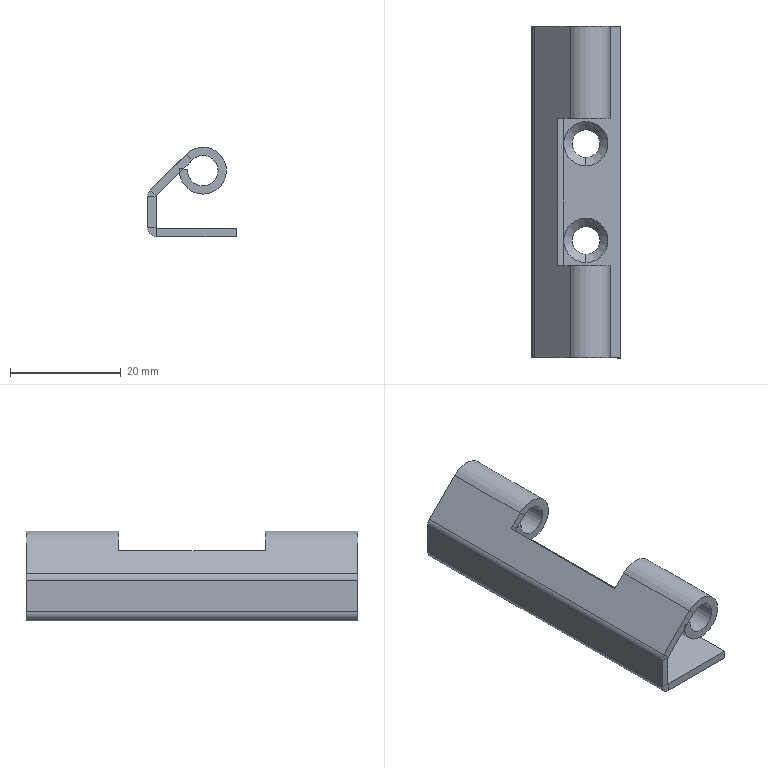Component | SolidWorks | AEBox-BoxHinge-3 | 1 solid | 38 faces | box 16 x 60 x 16.21 mm | volume 3571 mm3 | plane 26 | cylinder 8 | cone 4 | commonest cylinder face diameters 3.2 x2 0.2 x2 8.5 x2 5.5 x2
STEP:
#1=COLOUR_RGB('',0.7922,0.8196,0.9333);
#2=FILL_AREA_STYLE_COLOUR('',#1);
#3=FILL_AREA_STYLE('',(#2));
#4=SURFACE_STYLE_FILL_AREA(#3);
#5=SURFACE_SIDE_STYLE('',(#4));
#6=SURFACE_STYLE_USAGE(.BOTH.,#5);
#7=PRESENTATION_STYLE_ASSIGNMENT((#6));
#8=CARTESIAN_POINT('',(9.75,-14.031,37.663));
#9=VERTEX_POINT('',#8);
#10=CARTESIAN_POINT('',(9.75,-14.228,37.663));
#11=VERTEX_POINT('',#10);
#12=CARTESIAN_POINT('',(9.75,-14.129,37.663));
#13=DIRECTION('',(-0.,0.,-1.));
#14=DIRECTION('',(0.,-1.,0.));
#15=AXIS2_PLACEMENT_3D('',#12,#13,#14);
#16=CIRCLE('',#15,0.09843);
#17=EDGE_CURVE('',#9,#11,#16,.T.);
#18=ORIENTED_EDGE('',*,*,#17,.T.);
#19=CARTESIAN_POINT('',(9.75,-14.287,37.722));
#20=VERTEX_POINT('',#19);
#21=CARTESIAN_POINT('',(9.75,-14.287,37.722));
#22=DIRECTION('',(-0.,-0.7071,0.7071));
#23=VECTOR('',#22,39.37);
#24=LINE('',#21,#23);
#25=EDGE_CURVE('',#11,#20,#24,.T.);
#26=ORIENTED_EDGE('',*,*,#25,.T.);
#27=CARTESIAN_POINT('',(9.75,-13.972,37.722));
#28=VERTEX_POINT('',#27);
#29=CARTESIAN_POINT('',(9.75,-14.129,37.722));
#30=DIRECTION('',(-0.,0.,-1.));
#31=DIRECTION('',(-0.,-1.,0.));
#32=AXIS2_PLACEMENT_3D('',#29,#30,#31);
#33=CIRCLE('',#32,0.1575);
#34=EDGE_CURVE('',#28,#20,#33,.T.);
#35=ORIENTED_EDGE('',*,*,#34,.F.);
#36=CARTESIAN_POINT('',(9.75,-13.972,37.722));
#37=DIRECTION('',(0.,0.7071,0.7071));
#38=VECTOR('',#37,39.37);
#39=LINE('',#36,#38);
#40=EDGE_CURVE('',#9,#28,#39,.T.);
#41=ORIENTED_EDGE('',*,*,#40,.F.);
#42=EDGE_LOOP('',(#18,#26,#35,#41));
#43=FACE_OUTER_BOUND('',#42,.T.);
#44=CARTESIAN_POINT('',(9.75,-14.129,37.722));
#45=DIRECTION('',(0.,-0.,1.));
#46=DIRECTION('',(0.,1.,0.));
#47=AXIS2_PLACEMENT_3D('',#44,#45,#46);
#48=CONICAL_SURFACE('',#47,0.1575,0.7854);
#49=ADVANCED_FACE('',(#43),#48,.F.);
#50=CARTESIAN_POINT('',(9.75,-13.342,37.663));
#51=VERTEX_POINT('',#50);
#52=CARTESIAN_POINT('',(9.75,-13.539,37.663));
#53=VERTEX_POINT('',#52);
#54=CARTESIAN_POINT('',(9.75,-13.44,37.663));
#55=DIRECTION('',(-0.,0.,-1.));
#56=DIRECTION('',(0.,-1.,0.));
#57=AXIS2_PLACEMENT_3D('',#54,#55,#56);
#58=CIRCLE('',#57,0.09843);
#59=EDGE_CURVE('',#51,#53,#58,.T.);
#60=ORIENTED_EDGE('',*,*,#59,.T.);
#61=CARTESIAN_POINT('',(9.75,-13.598,37.722));
#62=VERTEX_POINT('',#61);
#63=CARTESIAN_POINT('',(9.75,-13.598,37.722));
#64=DIRECTION('',(-0.,-0.7071,0.7071));
#65=VECTOR('',#64,39.37);
#66=LINE('',#63,#65);
#67=EDGE_CURVE('',#53,#62,#66,.T.);
#68=ORIENTED_EDGE('',*,*,#67,.T.);
#69=CARTESIAN_POINT('',(9.75,-13.283,37.722));
#70=VERTEX_POINT('',#69);
#71=CARTESIAN_POINT('',(9.75,-13.44,37.722));
#72=DIRECTION('',(-0.,0.,-1.));
#73=DIRECTION('',(-0.,-1.,0.));
#74=AXIS2_PLACEMENT_3D('',#71,#72,#73);
#75=CIRCLE('',#74,0.1575);
#76=EDGE_CURVE('',#70,#62,#75,.T.);
#77=ORIENTED_EDGE('',*,*,#76,.F.);
#78=CARTESIAN_POINT('',(9.75,-13.283,37.722));
#79=DIRECTION('',(0.,0.7071,0.7071));
#80=VECTOR('',#79,39.37);
#81=LINE('',#78,#80);
#82=EDGE_CURVE('',#51,#70,#81,.T.);
#83=ORIENTED_EDGE('',*,*,#82,.F.);
#84=EDGE_LOOP('',(#60,#68,#77,#83));
#85=FACE_OUTER_BOUND('',#84,.T.);
#86=CARTESIAN_POINT('',(9.75,-13.44,37.722));
#87=DIRECTION('',(0.,-0.,1.));
#88=DIRECTION('',(0.,1.,0.));
#89=AXIS2_PLACEMENT_3D('',#86,#87,#88);
#90=CONICAL_SURFACE('',#89,0.1575,0.7854);
#91=ADVANCED_FACE('',(#85),#90,.F.);
#92=CARTESIAN_POINT('',(9.68,-14.966,38.21));
#93=VERTEX_POINT('',#92);
#94=CARTESIAN_POINT('',(9.424,-14.966,37.955));
#95=VERTEX_POINT('',#94);
#96=CARTESIAN_POINT('',(9.423,-14.966,37.953));
#97=DIRECTION('',(-0.7071,0.,-0.7071));
#98=VECTOR('',#97,39.37);
#99=LINE('',#96,#98);
#100=EDGE_CURVE('',#93,#95,#99,.T.);
#101=ORIENTED_EDGE('',*,*,#100,.F.);
#102=CARTESIAN_POINT('',(9.638,-14.966,38.252));
#103=VERTEX_POINT('',#102);
#104=CARTESIAN_POINT('',(9.68,-14.966,38.21));
#105=DIRECTION('',(-0.7071,0.,0.7071));
#106=VECTOR('',#105,39.37);
#107=LINE('',#104,#106);
#108=EDGE_CURVE('',#93,#103,#107,.T.);
#109=ORIENTED_EDGE('',*,*,#108,.T.);
#110=CARTESIAN_POINT('',(9.382,-14.966,37.996));
#111=VERTEX_POINT('',#110);
#112=CARTESIAN_POINT('',(9.381,-14.966,37.995));
#113=DIRECTION('',(-0.7071,0.,-0.7071));
#114=VECTOR('',#113,39.37);
#115=LINE('',#112,#114);
#116=EDGE_CURVE('',#103,#111,#115,.T.);
#117=ORIENTED_EDGE('',*,*,#116,.T.);
#118=CARTESIAN_POINT('',(9.424,-14.966,37.955));
#119=DIRECTION('',(-0.7071,0.,0.7071));
#120=VECTOR('',#119,39.37);
#121=LINE('',#118,#120);
#122=EDGE_CURVE('',#95,#111,#121,.T.);
#123=ORIENTED_EDGE('',*,*,#122,.F.);
#124=EDGE_LOOP('',(#101,#109,#117,#123));
#125=FACE_OUTER_BOUND('',#124,.T.);
#126=CARTESIAN_POINT('',(9.381,-14.966,37.995));
#127=DIRECTION('',(-0.,-1.,-0.));
#128=DIRECTION('',(0.,-0.,1.));
#129=AXIS2_PLACEMENT_3D('',#126,#127,#128);
#130=PLANE('',#129);
#131=ADVANCED_FACE('',(#125),#130,.T.);
#132=CARTESIAN_POINT('',(9.423,-14.966,37.952));
#133=VERTEX_POINT('',#132);
#134=CARTESIAN_POINT('',(9.364,-14.966,37.952));
#135=VERTEX_POINT('',#134);
#136=CARTESIAN_POINT('',(9.423,-14.966,37.952));
#137=DIRECTION('',(-1.,0.,0.));
#138=VECTOR('',#137,39.37);
#139=LINE('',#136,#138);
#140=EDGE_CURVE('',#133,#135,#139,.T.);
#141=ORIENTED_EDGE('',*,*,#140,.T.);
#142=CARTESIAN_POINT('',(9.364,-14.966,37.726));
#143=VERTEX_POINT('',#142);
#144=CARTESIAN_POINT('',(9.364,-14.966,37.722));
#145=DIRECTION('',(-0.,-0.,1.));
#146=VECTOR('',#145,39.37);
#147=LINE('',#144,#146);
#148=EDGE_CURVE('',#143,#135,#147,.T.);
#149=ORIENTED_EDGE('',*,*,#148,.F.);
#150=CARTESIAN_POINT('',(9.423,-14.966,37.726));
#151=VERTEX_POINT('',#150);
#152=CARTESIAN_POINT('',(9.423,-14.966,37.726));
#153=DIRECTION('',(-1.,0.,-0.));
#154=VECTOR('',#153,39.37);
#155=LINE('',#152,#154);
#156=EDGE_CURVE('',#151,#143,#155,.T.);
#157=ORIENTED_EDGE('',*,*,#156,.F.);
#158=CARTESIAN_POINT('',(9.423,-14.966,37.978));
#159=DIRECTION('',(-0.,-0.,1.));
#160=VECTOR('',#159,39.37);
#161=LINE('',#158,#160);
#162=EDGE_CURVE('',#151,#133,#161,.T.);
#163=ORIENTED_EDGE('',*,*,#162,.T.);
#164=EDGE_LOOP('',(#141,#149,#157,#163));
#165=FACE_OUTER_BOUND('',#164,.T.);
#166=CARTESIAN_POINT('',(9.364,-14.966,37.978));
#167=DIRECTION('',(0.,1.,0.));
#168=DIRECTION('',(-0.,0.,-1.));
#169=AXIS2_PLACEMENT_3D('',#166,#167,#168);
#170=PLANE('',#169);
#171=ADVANCED_FACE('',(#165),#170,.F.);
#172=CARTESIAN_POINT('',(9.423,-12.604,37.952));
#173=VERTEX_POINT('',#172);
#174=CARTESIAN_POINT('',(9.364,-12.604,37.952));
#175=VERTEX_POINT('',#174);
#176=CARTESIAN_POINT('',(9.423,-12.604,37.952));
#177=DIRECTION('',(-1.,0.,0.));
#178=VECTOR('',#177,39.37);
#179=LINE('',#176,#178);
#180=EDGE_CURVE('',#173,#175,#179,.T.);
#181=ORIENTED_EDGE('',*,*,#180,.F.);
#182=CARTESIAN_POINT('',(9.423,-12.604,37.726));
#183=VERTEX_POINT('',#182);
#184=CARTESIAN_POINT('',(9.423,-12.604,37.722));
#185=DIRECTION('',(0.,0.,-1.));
#186=VECTOR('',#185,39.37);
#187=LINE('',#184,#186);
#188=EDGE_CURVE('',#173,#183,#187,.T.);
#189=ORIENTED_EDGE('',*,*,#188,.T.);
#190=CARTESIAN_POINT('',(9.364,-12.604,37.726));
#191=VERTEX_POINT('',#190);
#192=CARTESIAN_POINT('',(9.364,-12.604,37.726));
#193=DIRECTION('',(-1.,0.,-0.));
#194=VECTOR('',#193,39.37);
#195=LINE('',#192,#194);
#196=EDGE_CURVE('',#183,#191,#195,.T.);
#197=ORIENTED_EDGE('',*,*,#196,.T.);
#198=CARTESIAN_POINT('',(9.364,-12.604,37.722));
#199=DIRECTION('',(0.,0.,-1.));
#200=VECTOR('',#199,39.37);
#201=LINE('',#198,#200);
#202=EDGE_CURVE('',#175,#191,#201,.T.);
#203=ORIENTED_EDGE('',*,*,#202,.F.);
#204=EDGE_LOOP('',(#181,#189,#197,#203));
#205=FACE_OUTER_BOUND('',#204,.T.);
#206=CARTESIAN_POINT('',(9.364,-12.604,37.722));
#207=DIRECTION('',(-0.,-1.,-0.));
#208=DIRECTION('',(0.,-0.,1.));
#209=AXIS2_PLACEMENT_3D('',#206,#207,#208);
#210=PLANE('',#209);
#211=ADVANCED_FACE('',(#205),#210,.F.);
#212=CARTESIAN_POINT('',(9.364,-14.966,37.952));
#213=DIRECTION('',(0.,1.,0.));
#214=VECTOR('',#213,39.37);
#215=LINE('',#212,#214);
#216=EDGE_CURVE('',#135,#175,#215,.T.);
#217=ORIENTED_EDGE('',*,*,#216,.T.);
#218=ORIENTED_EDGE('',*,*,#202,.T.);
#219=CARTESIAN_POINT('',(9.364,-12.604,37.726));
#220=DIRECTION('',(0.,1.,0.));
#221=VECTOR('',#220,39.37);
#222=LINE('',#219,#221);
#223=EDGE_CURVE('',#143,#191,#222,.T.);
#224=ORIENTED_EDGE('',*,*,#223,.F.);
#225=ORIENTED_EDGE('',*,*,#148,.T.);
#226=EDGE_LOOP('',(#217,#218,#224,#225));
#227=FACE_OUTER_BOUND('',#226,.T.);
#228=CARTESIAN_POINT('',(9.364,-14.966,37.722));
#229=DIRECTION('',(1.,-0.,0.));
#230=DIRECTION('',(-0.,-0.,1.));
#231=AXIS2_PLACEMENT_3D('',#228,#229,#230);
#232=PLANE('',#231);
#233=ADVANCED_FACE('',(#227),#232,.F.);
#234=ORIENTED_EDGE('',*,*,#188,.F.);
#235=CARTESIAN_POINT('',(9.423,-14.966,37.952));
#236=DIRECTION('',(0.,1.,0.));
#237=VECTOR('',#236,39.37);
#238=LINE('',#235,#237);
#239=EDGE_CURVE('',#133,#173,#238,.T.);
#240=ORIENTED_EDGE('',*,*,#239,.F.);
#241=ORIENTED_EDGE('',*,*,#162,.F.);
#242=CARTESIAN_POINT('',(9.423,-12.604,37.726));
#243=DIRECTION('',(-0.,-1.,-0.));
#244=VECTOR('',#243,39.37);
#245=LINE('',#242,#244);
#246=EDGE_CURVE('',#183,#151,#245,.T.);
#247=ORIENTED_EDGE('',*,*,#246,.F.);
#248=EDGE_LOOP('',(#234,#240,#241,#247));
#249=FACE_OUTER_BOUND('',#248,.T.);
#250=CARTESIAN_POINT('',(9.423,-14.966,37.722));
#251=DIRECTION('',(1.,-0.,0.));
#252=DIRECTION('',(-0.,-0.,1.));
#253=AXIS2_PLACEMENT_3D('',#250,#251,#252);
#254=PLANE('',#253);
#255=ADVANCED_FACE('',(#249),#254,.T.);
#256=CARTESIAN_POINT('',(9.994,-14.966,37.722));
#257=VERTEX_POINT('',#256);
#258=CARTESIAN_POINT('',(9.427,-14.966,37.722));
#259=VERTEX_POINT('',#258);
#260=CARTESIAN_POINT('',(9.364,-14.966,37.722));
#261=DIRECTION('',(-1.,0.,0.));
#262=VECTOR('',#261,39.37);
#263=LINE('',#260,#262);
#264=EDGE_CURVE('',#257,#259,#263,.T.);
#265=ORIENTED_EDGE('',*,*,#264,.T.);
#266=CARTESIAN_POINT('',(9.427,-14.966,37.663));
#267=VERTEX_POINT('',#266);
#268=CARTESIAN_POINT('',(9.427,-14.966,37.722));
#269=DIRECTION('',(-0.,0.,-1.));
#270=VECTOR('',#269,39.37);
#271=LINE('',#268,#270);
#272=EDGE_CURVE('',#259,#267,#271,.T.);
#273=ORIENTED_EDGE('',*,*,#272,.T.);
#274=CARTESIAN_POINT('',(9.994,-14.966,37.663));
#275=VERTEX_POINT('',#274);
#276=CARTESIAN_POINT('',(9.364,-14.966,37.663));
#277=DIRECTION('',(-1.,0.,0.));
#278=VECTOR('',#277,39.37);
#279=LINE('',#276,#278);
#280=EDGE_CURVE('',#275,#267,#279,.T.);
#281=ORIENTED_EDGE('',*,*,#280,.F.);
#282=CARTESIAN_POINT('',(9.994,-14.966,37.722));
#283=DIRECTION('',(-0.,0.,-1.));
#284=VECTOR('',#283,39.37);
#285=LINE('',#282,#284);
#286=EDGE_CURVE('',#257,#275,#285,.T.);
#287=ORIENTED_EDGE('',*,*,#286,.F.);
#288=EDGE_LOOP('',(#265,#273,#281,#287));
#289=FACE_OUTER_BOUND('',#288,.T.);
#290=CARTESIAN_POINT('',(9.364,-14.966,37.722));
#291=DIRECTION('',(-0.,-1.,-0.));
#292=DIRECTION('',(-1.,0.,0.));
#293=AXIS2_PLACEMENT_3D('',#290,#291,#292);
#294=PLANE('',#293);
#295=ADVANCED_FACE('',(#289),#294,.T.);
#296=ORIENTED_EDGE('',*,*,#76,.T.);
#297=CARTESIAN_POINT('',(9.75,-13.44,37.722));
#298=DIRECTION('',(-0.,0.,-1.));
#299=DIRECTION('',(-0.,-1.,0.));
#300=AXIS2_PLACEMENT_3D('',#297,#298,#299);
#301=CIRCLE('',#300,0.1575);
#302=EDGE_CURVE('',#62,#70,#301,.T.);
#303=ORIENTED_EDGE('',*,*,#302,.T.);
#304=EDGE_LOOP('',(#296,#303));
#305=FACE_BOUND('',#304,.T.);
#306=ORIENTED_EDGE('',*,*,#34,.T.);
#307=CARTESIAN_POINT('',(9.75,-14.129,37.722));
#308=DIRECTION('',(-0.,0.,-1.));
#309=DIRECTION('',(-0.,-1.,0.));
#310=AXIS2_PLACEMENT_3D('',#307,#308,#309);
#311=CIRCLE('',#310,0.1575);
#312=EDGE_CURVE('',#20,#28,#311,.T.);
#313=ORIENTED_EDGE('',*,*,#312,.T.);
#314=EDGE_LOOP('',(#306,#313));
#315=FACE_BOUND('',#314,.T.);
#316=CARTESIAN_POINT('',(9.427,-12.604,37.722));
#317=VERTEX_POINT('',#316);
#318=CARTESIAN_POINT('',(9.427,-14.966,37.722));
#319=DIRECTION('',(0.,1.,0.));
#320=VECTOR('',#319,39.37);
#321=LINE('',#318,#320);
#322=EDGE_CURVE('',#259,#317,#321,.T.);
#323=ORIENTED_EDGE('',*,*,#322,.F.);
#324=ORIENTED_EDGE('',*,*,#264,.F.);
#325=CARTESIAN_POINT('',(9.994,-12.604,37.722));
#326=VERTEX_POINT('',#325);
#327=CARTESIAN_POINT('',(9.994,-12.604,37.722));
#328=DIRECTION('',(-0.,-1.,-0.));
#329=VECTOR('',#328,39.37);
#330=LINE('',#327,#329);
#331=EDGE_CURVE('',#326,#257,#330,.T.);
#332=ORIENTED_EDGE('',*,*,#331,.F.);
#333=CARTESIAN_POINT('',(9.364,-12.604,37.722));
#334=DIRECTION('',(1.,-0.,-0.));
#335=VECTOR('',#334,39.37);
#336=LINE('',#333,#335);
#337=EDGE_CURVE('',#317,#326,#336,.T.);
#338=ORIENTED_EDGE('',*,*,#337,.F.);
#339=EDGE_LOOP('',(#323,#324,#332,#338));
#340=FACE_OUTER_BOUND('',#339,.T.);
#341=CARTESIAN_POINT('',(9.994,-14.966,37.722));
#342=DIRECTION('',(-0.,0.,-1.));
#343=DIRECTION('',(-0.,-1.,-0.));
#344=AXIS2_PLACEMENT_3D('',#341,#342,#343);
#345=PLANE('',#344);
#346=ADVANCED_FACE('',(#305,#315,#340),#345,.F.);
#347=ORIENTED_EDGE('',*,*,#59,.F.);
#348=CARTESIAN_POINT('',(9.75,-13.44,37.663));
#349=DIRECTION('',(-0.,0.,-1.));
#350=DIRECTION('',(0.,-1.,0.));
#351=AXIS2_PLACEMENT_3D('',#348,#349,#350);
#352=CIRCLE('',#351,0.09843);
#353=EDGE_CURVE('',#53,#51,#352,.T.);
#354=ORIENTED_EDGE('',*,*,#353,.F.);
#355=EDGE_LOOP('',(#347,#354));
#356=FACE_BOUND('',#355,.T.);
#357=ORIENTED_EDGE('',*,*,#17,.F.);
#358=CARTESIAN_POINT('',(9.75,-14.129,37.663));
#359=DIRECTION('',(-0.,0.,-1.));
#360=DIRECTION('',(0.,-1.,0.));
#361=AXIS2_PLACEMENT_3D('',#358,#359,#360);
#362=CIRCLE('',#361,0.09843);
#363=EDGE_CURVE('',#11,#9,#362,.T.);
#364=ORIENTED_EDGE('',*,*,#363,.F.);
#365=EDGE_LOOP('',(#357,#364));
#366=FACE_BOUND('',#365,.T.);
#367=ORIENTED_EDGE('',*,*,#280,.T.);
#368=CARTESIAN_POINT('',(9.427,-12.604,37.663));
#369=VERTEX_POINT('',#368);
#370=CARTESIAN_POINT('',(9.427,-14.966,37.663));
#371=DIRECTION('',(0.,1.,0.));
#372=VECTOR('',#371,39.37);
#373=LINE('',#370,#372);
#374=EDGE_CURVE('',#267,#369,#373,.T.);
#375=ORIENTED_EDGE('',*,*,#374,.T.);
#376=CARTESIAN_POINT('',(9.994,-12.604,37.663));
#377=VERTEX_POINT('',#376);
#378=CARTESIAN_POINT('',(9.364,-12.604,37.663));
#379=DIRECTION('',(1.,-0.,-0.));
#380=VECTOR('',#379,39.37);
#381=LINE('',#378,#380);
#382=EDGE_CURVE('',#369,#377,#381,.T.);
#383=ORIENTED_EDGE('',*,*,#382,.T.);
#384=CARTESIAN_POINT('',(9.994,-12.604,37.663));
#385=DIRECTION('',(-0.,-1.,-0.));
#386=VECTOR('',#385,39.37);
#387=LINE('',#384,#386);
#388=EDGE_CURVE('',#377,#275,#387,.T.);
#389=ORIENTED_EDGE('',*,*,#388,.T.);
#390=EDGE_LOOP('',(#367,#375,#383,#389));
#391=FACE_OUTER_BOUND('',#390,.T.);
#392=CARTESIAN_POINT('',(9.994,-14.966,37.663));
#393=DIRECTION('',(-0.,0.,-1.));
#394=DIRECTION('',(-0.,-1.,-0.));
#395=AXIS2_PLACEMENT_3D('',#392,#393,#394);
#396=PLANE('',#395);
#397=ADVANCED_FACE('',(#356,#366,#391),#396,.T.);
#398=ORIENTED_EDGE('',*,*,#388,.F.);
#399=CARTESIAN_POINT('',(9.994,-12.604,37.722));
#400=DIRECTION('',(-0.,0.,-1.));
#401=VECTOR('',#400,39.37);
#402=LINE('',#399,#401);
#403=EDGE_CURVE('',#326,#377,#402,.T.);
#404=ORIENTED_EDGE('',*,*,#403,.F.);
#405=ORIENTED_EDGE('',*,*,#331,.T.);
#406=ORIENTED_EDGE('',*,*,#286,.T.);
#407=EDGE_LOOP('',(#398,#404,#405,#406));
#408=FACE_OUTER_BOUND('',#407,.T.);
#409=CARTESIAN_POINT('',(9.994,-12.604,37.722));
#410=DIRECTION('',(1.,-0.,-0.));
#411=DIRECTION('',(0.,-0.,1.));
#412=AXIS2_PLACEMENT_3D('',#409,#410,#411);
#413=PLANE('',#412);
#414=ADVANCED_FACE('',(#408),#413,.T.);
#415=CARTESIAN_POINT('',(9.427,-12.604,37.722));
#416=DIRECTION('',(-0.,0.,-1.));
#417=VECTOR('',#416,39.37);
#418=LINE('',#415,#417);
#419=EDGE_CURVE('',#317,#369,#418,.T.);
#420=ORIENTED_EDGE('',*,*,#419,.F.);
#421=ORIENTED_EDGE('',*,*,#337,.T.);
#422=ORIENTED_EDGE('',*,*,#403,.T.);
#423=ORIENTED_EDGE('',*,*,#382,.F.);
#424=EDGE_LOOP('',(#420,#421,#422,#423));
#425=FACE_OUTER_BOUND('',#424,.T.);
#426=CARTESIAN_POINT('',(9.364,-12.604,37.722));
#427=DIRECTION('',(0.,1.,0.));
#428=DIRECTION('',(1.,-0.,-0.));
#429=AXIS2_PLACEMENT_3D('',#426,#427,#428);
#430=PLANE('',#429);
#431=ADVANCED_FACE('',(#425),#430,.T.);
#432=ORIENTED_EDGE('',*,*,#196,.F.);
#433=CARTESIAN_POINT('',(9.427,-12.604,37.726));
#434=DIRECTION('',(0.,1.,0.));
#435=DIRECTION('',(0.,0.,1.));
#436=AXIS2_PLACEMENT_3D('',#433,#434,#435);
#437=CIRCLE('',#436,0.003937);
#438=EDGE_CURVE('',#317,#183,#437,.T.);
#439=ORIENTED_EDGE('',*,*,#438,.F.);
#440=ORIENTED_EDGE('',*,*,#419,.T.);
#441=CARTESIAN_POINT('',(9.427,-12.604,37.726));
#442=DIRECTION('',(0.,1.,0.));
#443=DIRECTION('',(0.,0.,1.));
#444=AXIS2_PLACEMENT_3D('',#441,#442,#443);
#445=CIRCLE('',#444,0.06299);
#446=EDGE_CURVE('',#369,#191,#445,.T.);
#447=ORIENTED_EDGE('',*,*,#446,.T.);
#448=EDGE_LOOP('',(#432,#439,#440,#447));
#449=FACE_OUTER_BOUND('',#448,.T.);
#450=CARTESIAN_POINT('',(9.427,-12.604,37.726));
#451=DIRECTION('',(0.,1.,0.));
#452=DIRECTION('',(-0.,0.,-1.));
#453=AXIS2_PLACEMENT_3D('',#450,#451,#452);
#454=PLANE('',#453);
#455=ADVANCED_FACE('',(#449),#454,.T.);
#456=CARTESIAN_POINT('',(9.427,-14.966,37.726));
#457=DIRECTION('',(-0.,-1.,-0.));
#458=DIRECTION('',(0.,0.,1.));
#459=AXIS2_PLACEMENT_3D('',#456,#457,#458);
#460=CIRCLE('',#459,0.003937);
#461=EDGE_CURVE('',#151,#259,#460,.T.);
#462=ORIENTED_EDGE('',*,*,#461,.F.);
#463=ORIENTED_EDGE('',*,*,#156,.T.);
#464=CARTESIAN_POINT('',(9.427,-14.966,37.726));
#465=DIRECTION('',(-0.,-1.,-0.));
#466=DIRECTION('',(0.,0.,1.));
#467=AXIS2_PLACEMENT_3D('',#464,#465,#466);
#468=CIRCLE('',#467,0.06299);
#469=EDGE_CURVE('',#143,#267,#468,.T.);
#470=ORIENTED_EDGE('',*,*,#469,.T.);
#471=ORIENTED_EDGE('',*,*,#272,.F.);
#472=EDGE_LOOP('',(#462,#463,#470,#471));
#473=FACE_OUTER_BOUND('',#472,.T.);
#474=CARTESIAN_POINT('',(9.427,-14.966,37.726));
#475=DIRECTION('',(0.,1.,0.));
#476=DIRECTION('',(-0.,0.,-1.));
#477=AXIS2_PLACEMENT_3D('',#474,#475,#476);
#478=PLANE('',#477);
#479=ADVANCED_FACE('',(#473),#478,.F.);
#480=ORIENTED_EDGE('',*,*,#374,.F.);
#481=ORIENTED_EDGE('',*,*,#469,.F.);
#482=ORIENTED_EDGE('',*,*,#223,.T.);
#483=ORIENTED_EDGE('',*,*,#446,.F.);
#484=EDGE_LOOP('',(#480,#481,#482,#483));
#485=FACE_OUTER_BOUND('',#484,.T.);
#486=CARTESIAN_POINT('',(9.427,-14.966,37.726));
#487=DIRECTION('',(-0.,-1.,-0.));
#488=DIRECTION('',(-1.,0.,0.));
#489=AXIS2_PLACEMENT_3D('',#486,#487,#488);
#490=CYLINDRICAL_SURFACE('',#489,0.06299);
#491=ADVANCED_FACE('',(#485),#490,.T.);
#492=ORIENTED_EDGE('',*,*,#322,.T.);
#493=ORIENTED_EDGE('',*,*,#438,.T.);
#494=ORIENTED_EDGE('',*,*,#246,.T.);
#495=ORIENTED_EDGE('',*,*,#461,.T.);
#496=EDGE_LOOP('',(#492,#493,#494,#495));
#497=FACE_OUTER_BOUND('',#496,.T.);
#498=CARTESIAN_POINT('',(9.427,-14.966,37.726));
#499=DIRECTION('',(-0.,-1.,-0.));
#500=DIRECTION('',(-1.,0.,0.));
#501=AXIS2_PLACEMENT_3D('',#498,#499,#500);
#502=CYLINDRICAL_SURFACE('',#501,0.003937);
#503=ADVANCED_FACE('',(#497),#502,.F.);
#504=CARTESIAN_POINT('',(9.424,-12.604,37.955));
#505=VERTEX_POINT('',#504);
#506=CARTESIAN_POINT('',(9.382,-12.604,37.996));
#507=VERTEX_POINT('',#506);
#508=CARTESIAN_POINT('',(9.382,-12.604,37.996));
#509=DIRECTION('',(-0.7071,0.,0.7071));
#510=VECTOR('',#509,39.37);
#511=LINE('',#508,#510);
#512=EDGE_CURVE('',#505,#507,#511,.T.);
#513=ORIENTED_EDGE('',*,*,#512,.F.);
#514=CARTESIAN_POINT('',(9.427,-12.604,37.952));
#515=DIRECTION('',(0.,1.,0.));
#516=DIRECTION('',(0.,0.,1.));
#517=AXIS2_PLACEMENT_3D('',#514,#515,#516);
#518=CIRCLE('',#517,0.003937);
#519=EDGE_CURVE('',#173,#505,#518,.T.);
#520=ORIENTED_EDGE('',*,*,#519,.F.);
#521=ORIENTED_EDGE('',*,*,#180,.T.);
#522=CARTESIAN_POINT('',(9.427,-12.604,37.952));
#523=DIRECTION('',(0.,1.,0.));
#524=DIRECTION('',(0.,0.,1.));
#525=AXIS2_PLACEMENT_3D('',#522,#523,#524);
#526=CIRCLE('',#525,0.06299);
#527=EDGE_CURVE('',#175,#507,#526,.T.);
#528=ORIENTED_EDGE('',*,*,#527,.T.);
#529=EDGE_LOOP('',(#513,#520,#521,#528));
#530=FACE_OUTER_BOUND('',#529,.T.);
#531=CARTESIAN_POINT('',(9.427,-12.604,37.952));
#532=DIRECTION('',(0.,1.,0.));
#533=DIRECTION('',(-0.,0.,-1.));
#534=AXIS2_PLACEMENT_3D('',#531,#532,#533);
#535=PLANE('',#534);
#536=ADVANCED_FACE('',(#530),#535,.T.);
#537=CARTESIAN_POINT('',(9.427,-14.966,37.952));
#538=DIRECTION('',(-0.,-1.,-0.));
#539=DIRECTION('',(0.,0.,1.));
#540=AXIS2_PLACEMENT_3D('',#537,#538,#539);
#541=CIRCLE('',#540,0.003937);
#542=EDGE_CURVE('',#95,#133,#541,.T.);
#543=ORIENTED_EDGE('',*,*,#542,.F.);
#544=ORIENTED_EDGE('',*,*,#122,.T.);
#545=CARTESIAN_POINT('',(9.427,-14.966,37.952));
#546=DIRECTION('',(-0.,-1.,-0.));
#547=DIRECTION('',(0.,0.,1.));
#548=AXIS2_PLACEMENT_3D('',#545,#546,#547);
#549=CIRCLE('',#548,0.06299);
#550=EDGE_CURVE('',#111,#135,#549,.T.);
#551=ORIENTED_EDGE('',*,*,#550,.T.);
#552=ORIENTED_EDGE('',*,*,#140,.F.);
#553=EDGE_LOOP('',(#543,#544,#551,#552));
#554=FACE_OUTER_BOUND('',#553,.T.);
#555=CARTESIAN_POINT('',(9.427,-14.966,37.952));
#556=DIRECTION('',(0.,1.,0.));
#557=DIRECTION('',(-0.,0.,-1.));
#558=AXIS2_PLACEMENT_3D('',#555,#556,#557);
#559=PLANE('',#558);
#560=ADVANCED_FACE('',(#554),#559,.F.);
#561=ORIENTED_EDGE('',*,*,#216,.F.);
#562=ORIENTED_EDGE('',*,*,#550,.F.);
#563=CARTESIAN_POINT('',(9.382,-14.966,37.996));
#564=DIRECTION('',(-0.,-1.,-0.));
#565=VECTOR('',#564,39.37);
#566=LINE('',#563,#565);
#567=EDGE_CURVE('',#507,#111,#566,.T.);
#568=ORIENTED_EDGE('',*,*,#567,.F.);
#569=ORIENTED_EDGE('',*,*,#527,.F.);
#570=EDGE_LOOP('',(#561,#562,#568,#569));
#571=FACE_OUTER_BOUND('',#570,.T.);
#572=CARTESIAN_POINT('',(9.427,-14.966,37.952));
#573=DIRECTION('',(-0.,-1.,-0.));
#574=DIRECTION('',(-0.7071,0.,0.7071));
#575=AXIS2_PLACEMENT_3D('',#572,#573,#574);
#576=CYLINDRICAL_SURFACE('',#575,0.06299);
#577=ADVANCED_FACE('',(#571),#576,.T.);
#578=ORIENTED_EDGE('',*,*,#239,.T.);
#579=ORIENTED_EDGE('',*,*,#519,.T.);
#580=CARTESIAN_POINT('',(9.424,-12.604,37.955));
#581=DIRECTION('',(-0.,-1.,-0.));
#582=VECTOR('',#581,39.37);
#583=LINE('',#580,#582);
#584=EDGE_CURVE('',#505,#95,#583,.T.);
#585=ORIENTED_EDGE('',*,*,#584,.T.);
#586=ORIENTED_EDGE('',*,*,#542,.T.);
#587=EDGE_LOOP('',(#578,#579,#585,#586));
#588=FACE_OUTER_BOUND('',#587,.T.);
#589=CARTESIAN_POINT('',(9.427,-14.966,37.952));
#590=DIRECTION('',(-0.,-1.,-0.));
#591=DIRECTION('',(-0.7071,0.,0.7071));
#592=AXIS2_PLACEMENT_3D('',#589,#590,#591);
#593=CYLINDRICAL_SURFACE('',#592,0.003937);
#594=ADVANCED_FACE('',(#588),#593,.F.);
#595=CARTESIAN_POINT('',(9.68,-12.604,38.21));
#596=VERTEX_POINT('',#595);
#597=CARTESIAN_POINT('',(9.638,-12.604,38.252));
#598=VERTEX_POINT('',#597);
#599=CARTESIAN_POINT('',(9.68,-12.604,38.21));
#600=DIRECTION('',(-0.7071,0.,0.7071));
#601=VECTOR('',#600,39.37);
#602=LINE('',#599,#601);
#603=EDGE_CURVE('',#596,#598,#602,.T.);
#604=ORIENTED_EDGE('',*,*,#603,.F.);
#605=CARTESIAN_POINT('',(9.423,-12.604,37.953));
#606=DIRECTION('',(0.7071,-0.,0.7071));
#607=VECTOR('',#606,39.37);
#608=LINE('',#605,#607);
#609=EDGE_CURVE('',#505,#596,#608,.T.);
#610=ORIENTED_EDGE('',*,*,#609,.F.);
#611=ORIENTED_EDGE('',*,*,#512,.T.);
#612=CARTESIAN_POINT('',(9.756,-12.604,38.37));
#613=DIRECTION('',(0.7071,-0.,0.7071));
#614=VECTOR('',#613,39.37);
#615=LINE('',#612,#614);
#616=EDGE_CURVE('',#507,#598,#615,.T.);
#617=ORIENTED_EDGE('',*,*,#616,.T.);
#618=EDGE_LOOP('',(#604,#610,#611,#617));
#619=FACE_OUTER_BOUND('',#618,.T.);
#620=CARTESIAN_POINT('',(9.756,-12.604,38.37));
#621=DIRECTION('',(0.,1.,0.));
#622=DIRECTION('',(-0.,0.,-1.));
#623=AXIS2_PLACEMENT_3D('',#620,#621,#622);
#624=PLANE('',#623);
#625=ADVANCED_FACE('',(#619),#624,.T.);
#626=CARTESIAN_POINT('',(9.638,-13.263,38.252));
#627=VERTEX_POINT('',#626);
#628=CARTESIAN_POINT('',(9.638,-13.263,38.252));
#629=DIRECTION('',(0.,1.,0.));
#630=VECTOR('',#629,39.37);
#631=LINE('',#628,#630);
#632=EDGE_CURVE('',#627,#598,#631,.T.);
#633=ORIENTED_EDGE('',*,*,#632,.T.);
#634=ORIENTED_EDGE('',*,*,#616,.F.);
#635=ORIENTED_EDGE('',*,*,#567,.T.);
#636=ORIENTED_EDGE('',*,*,#116,.F.);
#637=CARTESIAN_POINT('',(9.638,-14.306,38.252));
#638=VERTEX_POINT('',#637);
#639=CARTESIAN_POINT('',(9.638,-14.966,38.252));
#640=DIRECTION('',(0.,1.,0.));
#641=VECTOR('',#640,39.37);
#642=LINE('',#639,#641);
#643=EDGE_CURVE('',#103,#638,#642,.T.);
#644=ORIENTED_EDGE('',*,*,#643,.T.);
#645=CARTESIAN_POINT('',(9.548,-14.306,38.162));
#646=VERTEX_POINT('',#645);
#647=CARTESIAN_POINT('',(9.548,-14.306,38.162));
#648=DIRECTION('',(0.7071,-0.,0.7071));
#649=VECTOR('',#648,39.37);
#650=LINE('',#647,#649);
#651=EDGE_CURVE('',#646,#638,#650,.T.);
#652=ORIENTED_EDGE('',*,*,#651,.F.);
#653=CARTESIAN_POINT('',(9.548,-13.263,38.162));
#654=VERTEX_POINT('',#653);
#655=CARTESIAN_POINT('',(9.548,-13.263,38.162));
#656=DIRECTION('',(-0.,-1.,-0.));
#657=VECTOR('',#656,39.37);
#658=LINE('',#655,#657);
#659=EDGE_CURVE('',#654,#646,#658,.T.);
#660=ORIENTED_EDGE('',*,*,#659,.F.);
#661=CARTESIAN_POINT('',(9.966,-13.263,38.58));
#662=DIRECTION('',(-0.7071,0.,-0.7071));
#663=VECTOR('',#662,39.37);
#664=LINE('',#661,#663);
#665=EDGE_CURVE('',#627,#654,#664,.T.);
#666=ORIENTED_EDGE('',*,*,#665,.F.);
#667=EDGE_LOOP('',(#633,#634,#635,#636,#644,#652,#660,#666));
#668=FACE_OUTER_BOUND('',#667,.T.);
#669=CARTESIAN_POINT('',(9.381,-14.966,37.995));
#670=DIRECTION('',(-0.7071,0.,0.7071));
#671=DIRECTION('',(-0.7071,0.,-0.7071));
#672=AXIS2_PLACEMENT_3D('',#669,#670,#671);
#673=PLANE('',#672);
#674=ADVANCED_FACE('',(#668),#673,.T.);
#675=ORIENTED_EDGE('',*,*,#609,.T.);
#676=CARTESIAN_POINT('',(9.68,-13.263,38.21));
#677=VERTEX_POINT('',#676);
#678=CARTESIAN_POINT('',(9.68,-13.263,38.21));
#679=DIRECTION('',(0.,1.,0.));
#680=VECTOR('',#679,39.37);
#681=LINE('',#678,#680);
#682=EDGE_CURVE('',#677,#596,#681,.T.);
#683=ORIENTED_EDGE('',*,*,#682,.F.);
#684=CARTESIAN_POINT('',(9.589,-13.263,38.12));
#685=VERTEX_POINT('',#684);
#686=CARTESIAN_POINT('',(9.423,-13.263,37.953));
#687=DIRECTION('',(-0.7071,0.,-0.7071));
#688=VECTOR('',#687,39.37);
#689=LINE('',#686,#688);
#690=EDGE_CURVE('',#677,#685,#689,.T.);
#691=ORIENTED_EDGE('',*,*,#690,.T.);
#692=CARTESIAN_POINT('',(9.589,-14.306,38.12));
#693=VERTEX_POINT('',#692);
#694=CARTESIAN_POINT('',(9.589,-14.966,38.12));
#695=DIRECTION('',(-0.,-1.,-0.));
#696=VECTOR('',#695,39.37);
#697=LINE('',#694,#696);
#698=EDGE_CURVE('',#685,#693,#697,.T.);
#699=ORIENTED_EDGE('',*,*,#698,.T.);
#700=CARTESIAN_POINT('',(9.68,-14.306,38.21));
#701=VERTEX_POINT('',#700);
#702=CARTESIAN_POINT('',(9.423,-14.306,37.953));
#703=DIRECTION('',(0.7071,-0.,0.7071));
#704=VECTOR('',#703,39.37);
#705=LINE('',#702,#704);
#706=EDGE_CURVE('',#693,#701,#705,.T.);
#707=ORIENTED_EDGE('',*,*,#706,.T.);
#708=CARTESIAN_POINT('',(9.68,-14.966,38.21));
#709=DIRECTION('',(0.,1.,0.));
#710=VECTOR('',#709,39.37);
#711=LINE('',#708,#710);
#712=EDGE_CURVE('',#93,#701,#711,.T.);
#713=ORIENTED_EDGE('',*,*,#712,.F.);
#714=ORIENTED_EDGE('',*,*,#100,.T.);
#715=ORIENTED_EDGE('',*,*,#584,.F.);
#716=EDGE_LOOP('',(#675,#683,#691,#699,#707,#713,#714,#715));
#717=FACE_OUTER_BOUND('',#716,.T.);
#718=CARTESIAN_POINT('',(9.423,-14.966,37.953));
#719=DIRECTION('',(-0.7071,0.,0.7071));
#720=DIRECTION('',(-0.7071,0.,-0.7071));
#721=AXIS2_PLACEMENT_3D('',#718,#719,#720);
#722=PLANE('',#721);
#723=ADVANCED_FACE('',(#717),#722,.F.);
#724=CARTESIAN_POINT('',(9.826,-13.263,37.883));
#725=DIRECTION('',(-0.7071,0.,0.7071));
#726=VECTOR('',#725,39.37);
#727=LINE('',#724,#726);
#728=EDGE_CURVE('',#685,#654,#727,.T.);
#729=ORIENTED_EDGE('',*,*,#728,.T.);
#730=ORIENTED_EDGE('',*,*,#659,.T.);
#731=CARTESIAN_POINT('',(9.826,-14.306,37.883));
#732=DIRECTION('',(-0.7071,0.,0.7071));
#733=VECTOR('',#732,39.37);
#734=LINE('',#731,#733);
#735=EDGE_CURVE('',#693,#646,#734,.T.);
#736=ORIENTED_EDGE('',*,*,#735,.F.);
#737=ORIENTED_EDGE('',*,*,#698,.F.);
#738=EDGE_LOOP('',(#729,#730,#736,#737));
#739=FACE_OUTER_BOUND('',#738,.T.);
#740=CARTESIAN_POINT('',(9.826,-13.263,37.883));
#741=DIRECTION('',(-0.7071,0.,-0.7071));
#742=DIRECTION('',(0.7071,-0.,-0.7071));
#743=AXIS2_PLACEMENT_3D('',#740,#741,#742);
#744=PLANE('',#743);
#745=ADVANCED_FACE('',(#739),#744,.F.);
#746=ORIENTED_EDGE('',*,*,#651,.T.);
#747=CARTESIAN_POINT('',(9.68,-14.306,38.21));
#748=DIRECTION('',(-0.7071,0.,0.7071));
#749=VECTOR('',#748,39.37);
#750=LINE('',#747,#749);
#751=EDGE_CURVE('',#701,#638,#750,.T.);
#752=ORIENTED_EDGE('',*,*,#751,.F.);
#753=ORIENTED_EDGE('',*,*,#706,.F.);
#754=ORIENTED_EDGE('',*,*,#735,.T.);
#755=EDGE_LOOP('',(#746,#752,#753,#754));
#756=FACE_OUTER_BOUND('',#755,.T.);
#757=CARTESIAN_POINT('',(9.826,-14.306,37.883));
#758=DIRECTION('',(-0.,-1.,-0.));
#759=DIRECTION('',(0.,-0.,1.));
#760=AXIS2_PLACEMENT_3D('',#757,#758,#759);
#761=PLANE('',#760);
#762=ADVANCED_FACE('',(#756),#761,.F.);
#763=ORIENTED_EDGE('',*,*,#690,.F.);
#764=CARTESIAN_POINT('',(9.68,-13.263,38.21));
#765=DIRECTION('',(-0.7071,0.,0.7071));
#766=VECTOR('',#765,39.37);
#767=LINE('',#764,#766);
#768=EDGE_CURVE('',#677,#627,#767,.T.);
#769=ORIENTED_EDGE('',*,*,#768,.T.);
#770=ORIENTED_EDGE('',*,*,#665,.T.);
#771=ORIENTED_EDGE('',*,*,#728,.F.);
#772=EDGE_LOOP('',(#763,#769,#770,#771));
#773=FACE_OUTER_BOUND('',#772,.T.);
#774=CARTESIAN_POINT('',(10.244,-13.263,38.301));
#775=DIRECTION('',(0.,1.,0.));
#776=DIRECTION('',(-0.,0.,-1.));
#777=AXIS2_PLACEMENT_3D('',#774,#775,#776);
#778=PLANE('',#777);
#779=ADVANCED_FACE('',(#773),#778,.F.);
#780=CARTESIAN_POINT('',(9.648,-14.966,38.143));
#781=VERTEX_POINT('',#780);
#782=CARTESIAN_POINT('',(9.59,-14.966,38.148));
#783=VERTEX_POINT('',#782);
#784=CARTESIAN_POINT('',(9.648,-14.966,38.143));
#785=DIRECTION('',(-0.9962,0.,0.08716));
#786=VECTOR('',#785,39.37);
#787=LINE('',#784,#786);
#788=EDGE_CURVE('',#781,#783,#787,.T.);
#789=ORIENTED_EDGE('',*,*,#788,.F.);
#790=CARTESIAN_POINT('',(9.648,-14.306,38.143));
#791=VERTEX_POINT('',#790);
#792=CARTESIAN_POINT('',(9.648,-14.966,38.143));
#793=DIRECTION('',(-0.,-1.,-0.));
#794=VECTOR('',#793,39.37);
#795=LINE('',#792,#794);
#796=EDGE_CURVE('',#791,#781,#795,.T.);
#797=ORIENTED_EDGE('',*,*,#796,.F.);
#798=CARTESIAN_POINT('',(9.59,-14.306,38.148));
#799=VERTEX_POINT('',#798);
#800=CARTESIAN_POINT('',(9.648,-14.306,38.143));
#801=DIRECTION('',(-0.9962,0.,0.08716));
#802=VECTOR('',#801,39.37);
#803=LINE('',#800,#802);
#804=EDGE_CURVE('',#791,#799,#803,.T.);
#805=ORIENTED_EDGE('',*,*,#804,.T.);
#806=CARTESIAN_POINT('',(9.59,-14.966,38.148));
#807=DIRECTION('',(-0.,-1.,-0.));
#808=VECTOR('',#807,39.37);
#809=LINE('',#806,#808);
#810=EDGE_CURVE('',#799,#783,#809,.T.);
#811=ORIENTED_EDGE('',*,*,#810,.T.);
#812=EDGE_LOOP('',(#789,#797,#805,#811));
#813=FACE_OUTER_BOUND('',#812,.T.);
#814=CARTESIAN_POINT('',(9.648,-14.636,38.143));
#815=DIRECTION('',(-0.08716,0.,-0.9962));
#816=DIRECTION('',(-0.,-1.,-0.));
#817=AXIS2_PLACEMENT_3D('',#814,#815,#816);
#818=PLANE('',#817);
#819=ADVANCED_FACE('',(#813),#818,.F.);
#820=ORIENTED_EDGE('',*,*,#804,.F.);
#821=CARTESIAN_POINT('',(9.756,-14.306,38.134));
#822=DIRECTION('',(0.,1.,0.));
#823=DIRECTION('',(0.,0.,1.));
#824=AXIS2_PLACEMENT_3D('',#821,#822,#823);
#825=CIRCLE('',#824,0.1083);
#826=EDGE_CURVE('',#701,#791,#825,.T.);
#827=ORIENTED_EDGE('',*,*,#826,.F.);
#828=ORIENTED_EDGE('',*,*,#751,.T.);
#829=CARTESIAN_POINT('',(9.756,-14.306,38.134));
#830=DIRECTION('',(0.,1.,0.));
#831=DIRECTION('',(0.,0.,1.));
#832=AXIS2_PLACEMENT_3D('',#829,#830,#831);
#833=CIRCLE('',#832,0.1673);
#834=EDGE_CURVE('',#638,#799,#833,.T.);
#835=ORIENTED_EDGE('',*,*,#834,.T.);
#836=EDGE_LOOP('',(#820,#827,#828,#835));
#837=FACE_OUTER_BOUND('',#836,.T.);
#838=CARTESIAN_POINT('',(9.756,-14.306,38.134));
#839=DIRECTION('',(0.,1.,0.));
#840=DIRECTION('',(-0.,0.,-1.));
#841=AXIS2_PLACEMENT_3D('',#838,#839,#840);
#842=PLANE('',#841);
#843=ADVANCED_FACE('',(#837),#842,.T.);
#844=CARTESIAN_POINT('',(9.756,-14.966,38.134));
#845=DIRECTION('',(-0.,-1.,-0.));
#846=DIRECTION('',(0.,0.,1.));
#847=AXIS2_PLACEMENT_3D('',#844,#845,#846);
#848=CIRCLE('',#847,0.1083);
#849=EDGE_CURVE('',#781,#93,#848,.T.);
#850=ORIENTED_EDGE('',*,*,#849,.F.);
#851=ORIENTED_EDGE('',*,*,#788,.T.);
#852=CARTESIAN_POINT('',(9.756,-14.966,38.134));
#853=DIRECTION('',(-0.,-1.,-0.));
#854=DIRECTION('',(0.,0.,1.));
#855=AXIS2_PLACEMENT_3D('',#852,#853,#854);
#856=CIRCLE('',#855,0.1673);
#857=EDGE_CURVE('',#783,#103,#856,.T.);
#858=ORIENTED_EDGE('',*,*,#857,.T.);
#859=ORIENTED_EDGE('',*,*,#108,.F.);
#860=EDGE_LOOP('',(#850,#851,#858,#859));
#861=FACE_OUTER_BOUND('',#860,.T.);
#862=CARTESIAN_POINT('',(9.756,-14.966,38.134));
#863=DIRECTION('',(0.,1.,0.));
#864=DIRECTION('',(-0.,0.,-1.));
#865=AXIS2_PLACEMENT_3D('',#862,#863,#864);
#866=PLANE('',#865);
#867=ADVANCED_FACE('',(#861),#866,.F.);
#868=ORIENTED_EDGE('',*,*,#643,.F.);
#869=ORIENTED_EDGE('',*,*,#857,.F.);
#870=ORIENTED_EDGE('',*,*,#810,.F.);
#871=ORIENTED_EDGE('',*,*,#834,.F.);
#872=EDGE_LOOP('',(#868,#869,#870,#871));
#873=FACE_OUTER_BOUND('',#872,.T.);
#874=CARTESIAN_POINT('',(9.756,-14.966,38.134));
#875=DIRECTION('',(-0.,-1.,-0.));
#876=DIRECTION('',(-0.9962,0.,0.08716));
#877=AXIS2_PLACEMENT_3D('',#874,#875,#876);
#878=CYLINDRICAL_SURFACE('',#877,0.1673);
#879=ADVANCED_FACE('',(#873),#878,.T.);
#880=ORIENTED_EDGE('',*,*,#712,.T.);
#881=ORIENTED_EDGE('',*,*,#826,.T.);
#882=ORIENTED_EDGE('',*,*,#796,.T.);
#883=ORIENTED_EDGE('',*,*,#849,.T.);
#884=EDGE_LOOP('',(#880,#881,#882,#883));
#885=FACE_OUTER_BOUND('',#884,.T.);
#886=CARTESIAN_POINT('',(9.756,-14.966,38.134));
#887=DIRECTION('',(-0.,-1.,-0.));
#888=DIRECTION('',(-0.9962,0.,0.08716));
#889=AXIS2_PLACEMENT_3D('',#886,#887,#888);
#890=CYLINDRICAL_SURFACE('',#889,0.1083);
#891=ADVANCED_FACE('',(#885),#890,.F.);
#892=CARTESIAN_POINT('',(9.648,-13.263,38.143));
#893=VERTEX_POINT('',#892);
#894=CARTESIAN_POINT('',(9.59,-13.263,38.148));
#895=VERTEX_POINT('',#894);
#896=CARTESIAN_POINT('',(9.648,-13.263,38.143));
#897=DIRECTION('',(-0.9962,0.,0.08716));
#898=VECTOR('',#897,39.37);
#899=LINE('',#896,#898);
#900=EDGE_CURVE('',#893,#895,#899,.T.);
#901=ORIENTED_EDGE('',*,*,#900,.F.);
#902=CARTESIAN_POINT('',(9.648,-12.604,38.143));
#903=VERTEX_POINT('',#902);
#904=CARTESIAN_POINT('',(9.648,-13.263,38.143));
#905=DIRECTION('',(-0.,-1.,-0.));
#906=VECTOR('',#905,39.37);
#907=LINE('',#904,#906);
#908=EDGE_CURVE('',#903,#893,#907,.T.);
#909=ORIENTED_EDGE('',*,*,#908,.F.);
#910=CARTESIAN_POINT('',(9.59,-12.604,38.148));
#911=VERTEX_POINT('',#910);
#912=CARTESIAN_POINT('',(9.648,-12.604,38.143));
#913=DIRECTION('',(-0.9962,0.,0.08716));
#914=VECTOR('',#913,39.37);
#915=LINE('',#912,#914);
#916=EDGE_CURVE('',#903,#911,#915,.T.);
#917=ORIENTED_EDGE('',*,*,#916,.T.);
#918=CARTESIAN_POINT('',(9.59,-13.263,38.148));
#919=DIRECTION('',(-0.,-1.,-0.));
#920=VECTOR('',#919,39.37);
#921=LINE('',#918,#920);
#922=EDGE_CURVE('',#911,#895,#921,.T.);
#923=ORIENTED_EDGE('',*,*,#922,.T.);
#924=EDGE_LOOP('',(#901,#909,#917,#923));
#925=FACE_OUTER_BOUND('',#924,.T.);
#926=CARTESIAN_POINT('',(9.648,-12.933,38.143));
#927=DIRECTION('',(-0.08716,0.,-0.9962));
#928=DIRECTION('',(-0.,-1.,-0.));
#929=AXIS2_PLACEMENT_3D('',#926,#927,#928);
#930=PLANE('',#929);
#931=ADVANCED_FACE('',(#925),#930,.F.);
#932=ORIENTED_EDGE('',*,*,#916,.F.);
#933=CARTESIAN_POINT('',(9.756,-12.604,38.134));
#934=DIRECTION('',(0.,1.,0.));
#935=DIRECTION('',(-1.,0.,0.));
#936=AXIS2_PLACEMENT_3D('',#933,#934,#935);
#937=CIRCLE('',#936,0.1083);
#938=EDGE_CURVE('',#596,#903,#937,.T.);
#939=ORIENTED_EDGE('',*,*,#938,.F.);
#940=ORIENTED_EDGE('',*,*,#603,.T.);
#941=CARTESIAN_POINT('',(9.756,-12.604,38.134));
#942=DIRECTION('',(0.,1.,0.));
#943=DIRECTION('',(-1.,0.,0.));
#944=AXIS2_PLACEMENT_3D('',#941,#942,#943);
#945=CIRCLE('',#944,0.1673);
#946=EDGE_CURVE('',#598,#911,#945,.T.);
#947=ORIENTED_EDGE('',*,*,#946,.T.);
#948=EDGE_LOOP('',(#932,#939,#940,#947));
#949=FACE_OUTER_BOUND('',#948,.T.);
#950=CARTESIAN_POINT('',(9.756,-12.604,38.134));
#951=DIRECTION('',(0.,1.,0.));
#952=DIRECTION('',(1.,-0.,-0.));
#953=AXIS2_PLACEMENT_3D('',#950,#951,#952);
#954=PLANE('',#953);
#955=ADVANCED_FACE('',(#949),#954,.T.);
#956=CARTESIAN_POINT('',(9.756,-13.263,38.134));
#957=DIRECTION('',(-0.,-1.,-0.));
#958=DIRECTION('',(-1.,0.,0.));
#959=AXIS2_PLACEMENT_3D('',#956,#957,#958);
#960=CIRCLE('',#959,0.1083);
#961=EDGE_CURVE('',#893,#677,#960,.T.);
#962=ORIENTED_EDGE('',*,*,#961,.F.);
#963=ORIENTED_EDGE('',*,*,#900,.T.);
#964=CARTESIAN_POINT('',(9.756,-13.263,38.134));
#965=DIRECTION('',(-0.,-1.,-0.));
#966=DIRECTION('',(-1.,0.,0.));
#967=AXIS2_PLACEMENT_3D('',#964,#965,#966);
#968=CIRCLE('',#967,0.1673);
#969=EDGE_CURVE('',#895,#627,#968,.T.);
#970=ORIENTED_EDGE('',*,*,#969,.T.);
#971=ORIENTED_EDGE('',*,*,#768,.F.);
#972=EDGE_LOOP('',(#962,#963,#970,#971));
#973=FACE_OUTER_BOUND('',#972,.T.);
#974=CARTESIAN_POINT('',(9.756,-13.263,38.134));
#975=DIRECTION('',(0.,1.,0.));
#976=DIRECTION('',(1.,-0.,-0.));
#977=AXIS2_PLACEMENT_3D('',#974,#975,#976);
#978=PLANE('',#977);
#979=ADVANCED_FACE('',(#973),#978,.F.);
#980=ORIENTED_EDGE('',*,*,#632,.F.);
#981=ORIENTED_EDGE('',*,*,#969,.F.);
#982=ORIENTED_EDGE('',*,*,#922,.F.);
#983=ORIENTED_EDGE('',*,*,#946,.F.);
#984=EDGE_LOOP('',(#980,#981,#982,#983));
#985=FACE_OUTER_BOUND('',#984,.T.);
#986=CARTESIAN_POINT('',(9.756,-13.263,38.134));
#987=DIRECTION('',(-0.,-1.,-0.));
#988=DIRECTION('',(-0.9962,0.,0.08716));
#989=AXIS2_PLACEMENT_3D('',#986,#987,#988);
#990=CYLINDRICAL_SURFACE('',#989,0.1673);
#991=ADVANCED_FACE('',(#985),#990,.T.);
#992=ORIENTED_EDGE('',*,*,#682,.T.);
#993=ORIENTED_EDGE('',*,*,#938,.T.);
#994=ORIENTED_EDGE('',*,*,#908,.T.);
#995=ORIENTED_EDGE('',*,*,#961,.T.);
#996=EDGE_LOOP('',(#992,#993,#994,#995));
#997=FACE_OUTER_BOUND('',#996,.T.);
#998=CARTESIAN_POINT('',(9.756,-13.263,38.134));
#999=DIRECTION('',(-0.,-1.,-0.));
#1000=DIRECTION('',(-0.9962,0.,0.08716));
#1001=AXIS2_PLACEMENT_3D('',#998,#999,#1000);
#1002=CYLINDRICAL_SURFACE('',#1001,0.1083);
#1003=ADVANCED_FACE('',(#997),#1002,.F.);
#1004=ORIENTED_EDGE('',*,*,#67,.F.);
#1005=ORIENTED_EDGE('',*,*,#353,.T.);
#1006=ORIENTED_EDGE('',*,*,#82,.T.);
#1007=ORIENTED_EDGE('',*,*,#302,.F.);
#1008=EDGE_LOOP('',(#1004,#1005,#1006,#1007));
#1009=FACE_OUTER_BOUND('',#1008,.T.);
#1010=CARTESIAN_POINT('',(9.75,-13.44,37.722));
#1011=DIRECTION('',(0.,-0.,1.));
#1012=DIRECTION('',(0.,1.,0.));
#1013=AXIS2_PLACEMENT_3D('',#1010,#1011,#1012);
#1014=CONICAL_SURFACE('',#1013,0.1575,0.7854);
#1015=ADVANCED_FACE('',(#1009),#1014,.F.);
#1016=ORIENTED_EDGE('',*,*,#25,.F.);
#1017=ORIENTED_EDGE('',*,*,#363,.T.);
#1018=ORIENTED_EDGE('',*,*,#40,.T.);
#1019=ORIENTED_EDGE('',*,*,#312,.F.);
#1020=EDGE_LOOP('',(#1016,#1017,#1018,#1019));
#1021=FACE_OUTER_BOUND('',#1020,.T.);
#1022=CARTESIAN_POINT('',(9.75,-14.129,37.722));
#1023=DIRECTION('',(0.,-0.,1.));
#1024=DIRECTION('',(0.,1.,0.));
#1025=AXIS2_PLACEMENT_3D('',#1022,#1023,#1024);
#1026=CONICAL_SURFACE('',#1025,0.1575,0.7854);
#1027=ADVANCED_FACE('',(#1021),#1026,.F.);
#1028=CLOSED_SHELL('',(#49,#91,#131,#171,#211,#233,#255,#295,#346,#397,#414,#431,#455,#479,#491,#503,#536,#560,#577,#594,#625,#674,#723,#745,#762,#779,#819,#843,#867,#879,#891,#931,#955,#979,#991,#1003,#1015,#1027));
#1029=MANIFOLD_SOLID_BREP('',#1028);
#1030=STYLED_ITEM('',(#7),#1029);
#1031=(LENGTH_UNIT()NAMED_UNIT(*)SI_UNIT($,.METRE.));
#1032=LENGTH_MEASURE_WITH_UNIT(LENGTH_MEASURE(0.0254),#1031);
#1033=DIMENSIONAL_EXPONENTS(1.,0.,0.,0.,0.,0.,0.);
#1034=(CONVERSION_BASED_UNIT('',#1032)LENGTH_UNIT()NAMED_UNIT(#1033));
#1035=UNCERTAINTY_MEASURE_WITH_UNIT(LENGTH_MEASURE(0.00001),#1034,'','');
#1036=(NAMED_UNIT(*)PLANE_ANGLE_UNIT()SI_UNIT($,.RADIAN.));
#1037=(NAMED_UNIT(*)SI_UNIT($,.STERADIAN.)SOLID_ANGLE_UNIT());
#1038=(GEOMETRIC_REPRESENTATION_CONTEXT(3)GLOBAL_UNCERTAINTY_ASSIGNED_CONTEXT((#1035))GLOBAL_UNIT_ASSIGNED_CONTEXT((#1034,#1036,#1037))REPRESENTATION_CONTEXT('',''));
#1039=MECHANICAL_DESIGN_GEOMETRIC_PRESENTATION_REPRESENTATION('',(#1030),#1038);
#1040=PRESENTATION_LAYER_ASSIGNMENT('','',(#1030));
#1041=CARTESIAN_POINT('',(0.,0.,0.));
#1042=DIRECTION('',(0.,0.,1.));
#1043=DIRECTION('',(1.,0.,0.));
#1044=AXIS2_PLACEMENT_3D('',#1041,#1042,#1043);
#1045=(LENGTH_UNIT()NAMED_UNIT(*)SI_UNIT($,.METRE.));
#1046=LENGTH_MEASURE_WITH_UNIT(LENGTH_MEASURE(0.0254),#1045);
#1047=DIMENSIONAL_EXPONENTS(1.,0.,0.,0.,0.,0.,0.);
#1048=(CONVERSION_BASED_UNIT('',#1046)LENGTH_UNIT()NAMED_UNIT(#1047));
#1049=UNCERTAINTY_MEASURE_WITH_UNIT(LENGTH_MEASURE(0.00001),#1048,'','');
#1050=(NAMED_UNIT(*)PLANE_ANGLE_UNIT()SI_UNIT($,.RADIAN.));
#1051=(NAMED_UNIT(*)SI_UNIT($,.STERADIAN.)SOLID_ANGLE_UNIT());
#1052=(GEOMETRIC_REPRESENTATION_CONTEXT(3)GLOBAL_UNCERTAINTY_ASSIGNED_CONTEXT((#1049))GLOBAL_UNIT_ASSIGNED_CONTEXT((#1048,#1050,#1051))REPRESENTATION_CONTEXT('',''));
#1053=ADVANCED_BREP_SHAPE_REPRESENTATION('',(#1029,#1044),#1052);